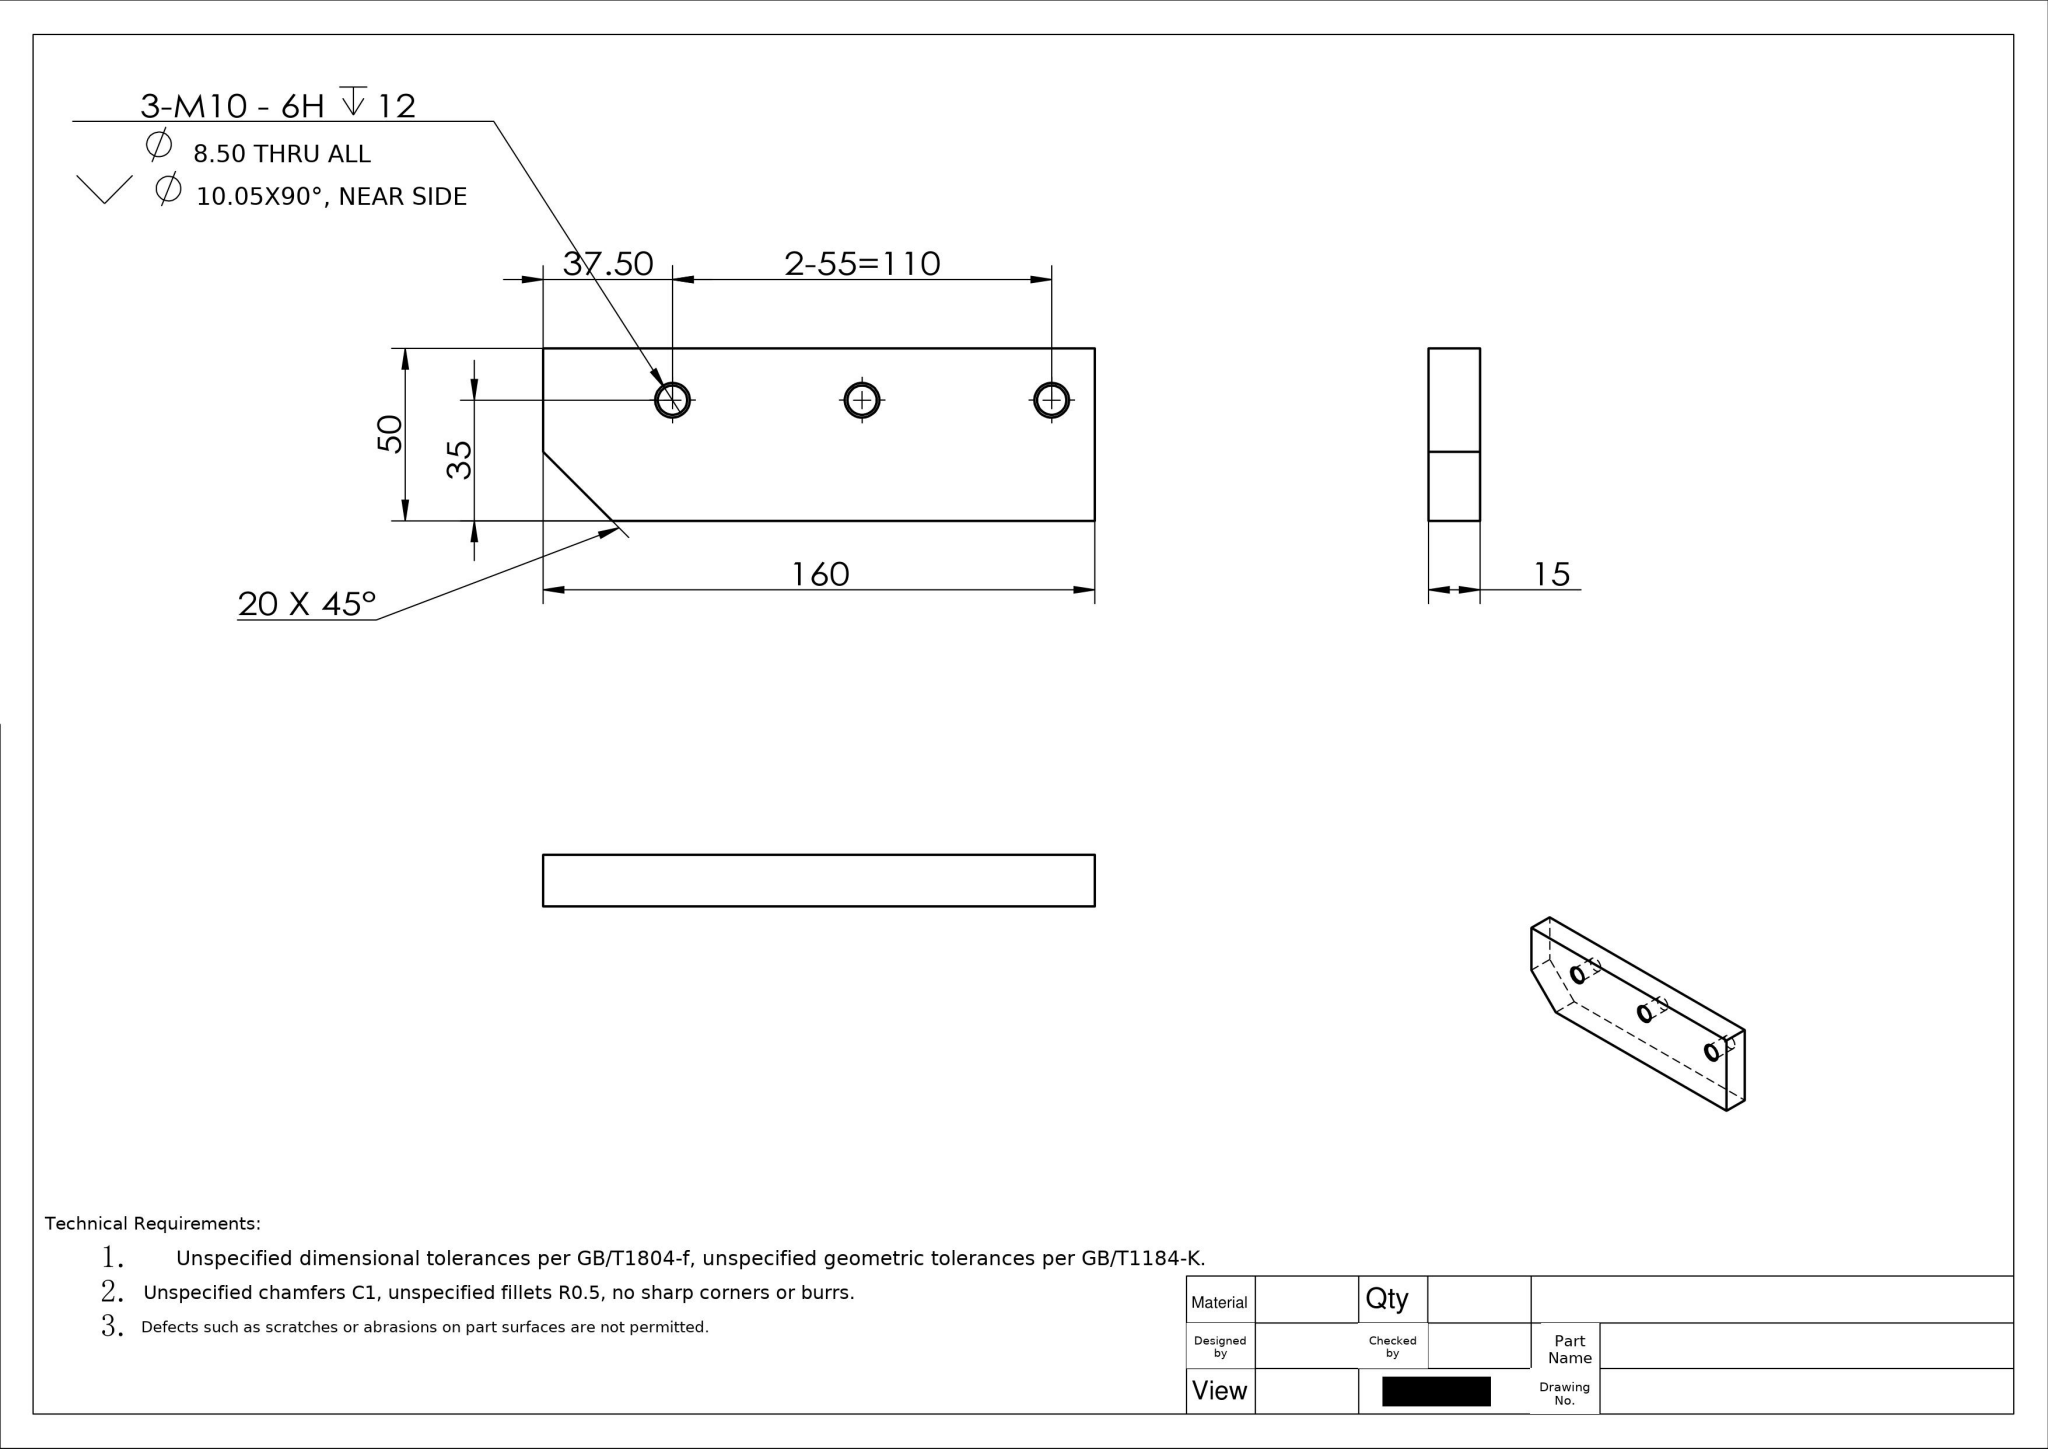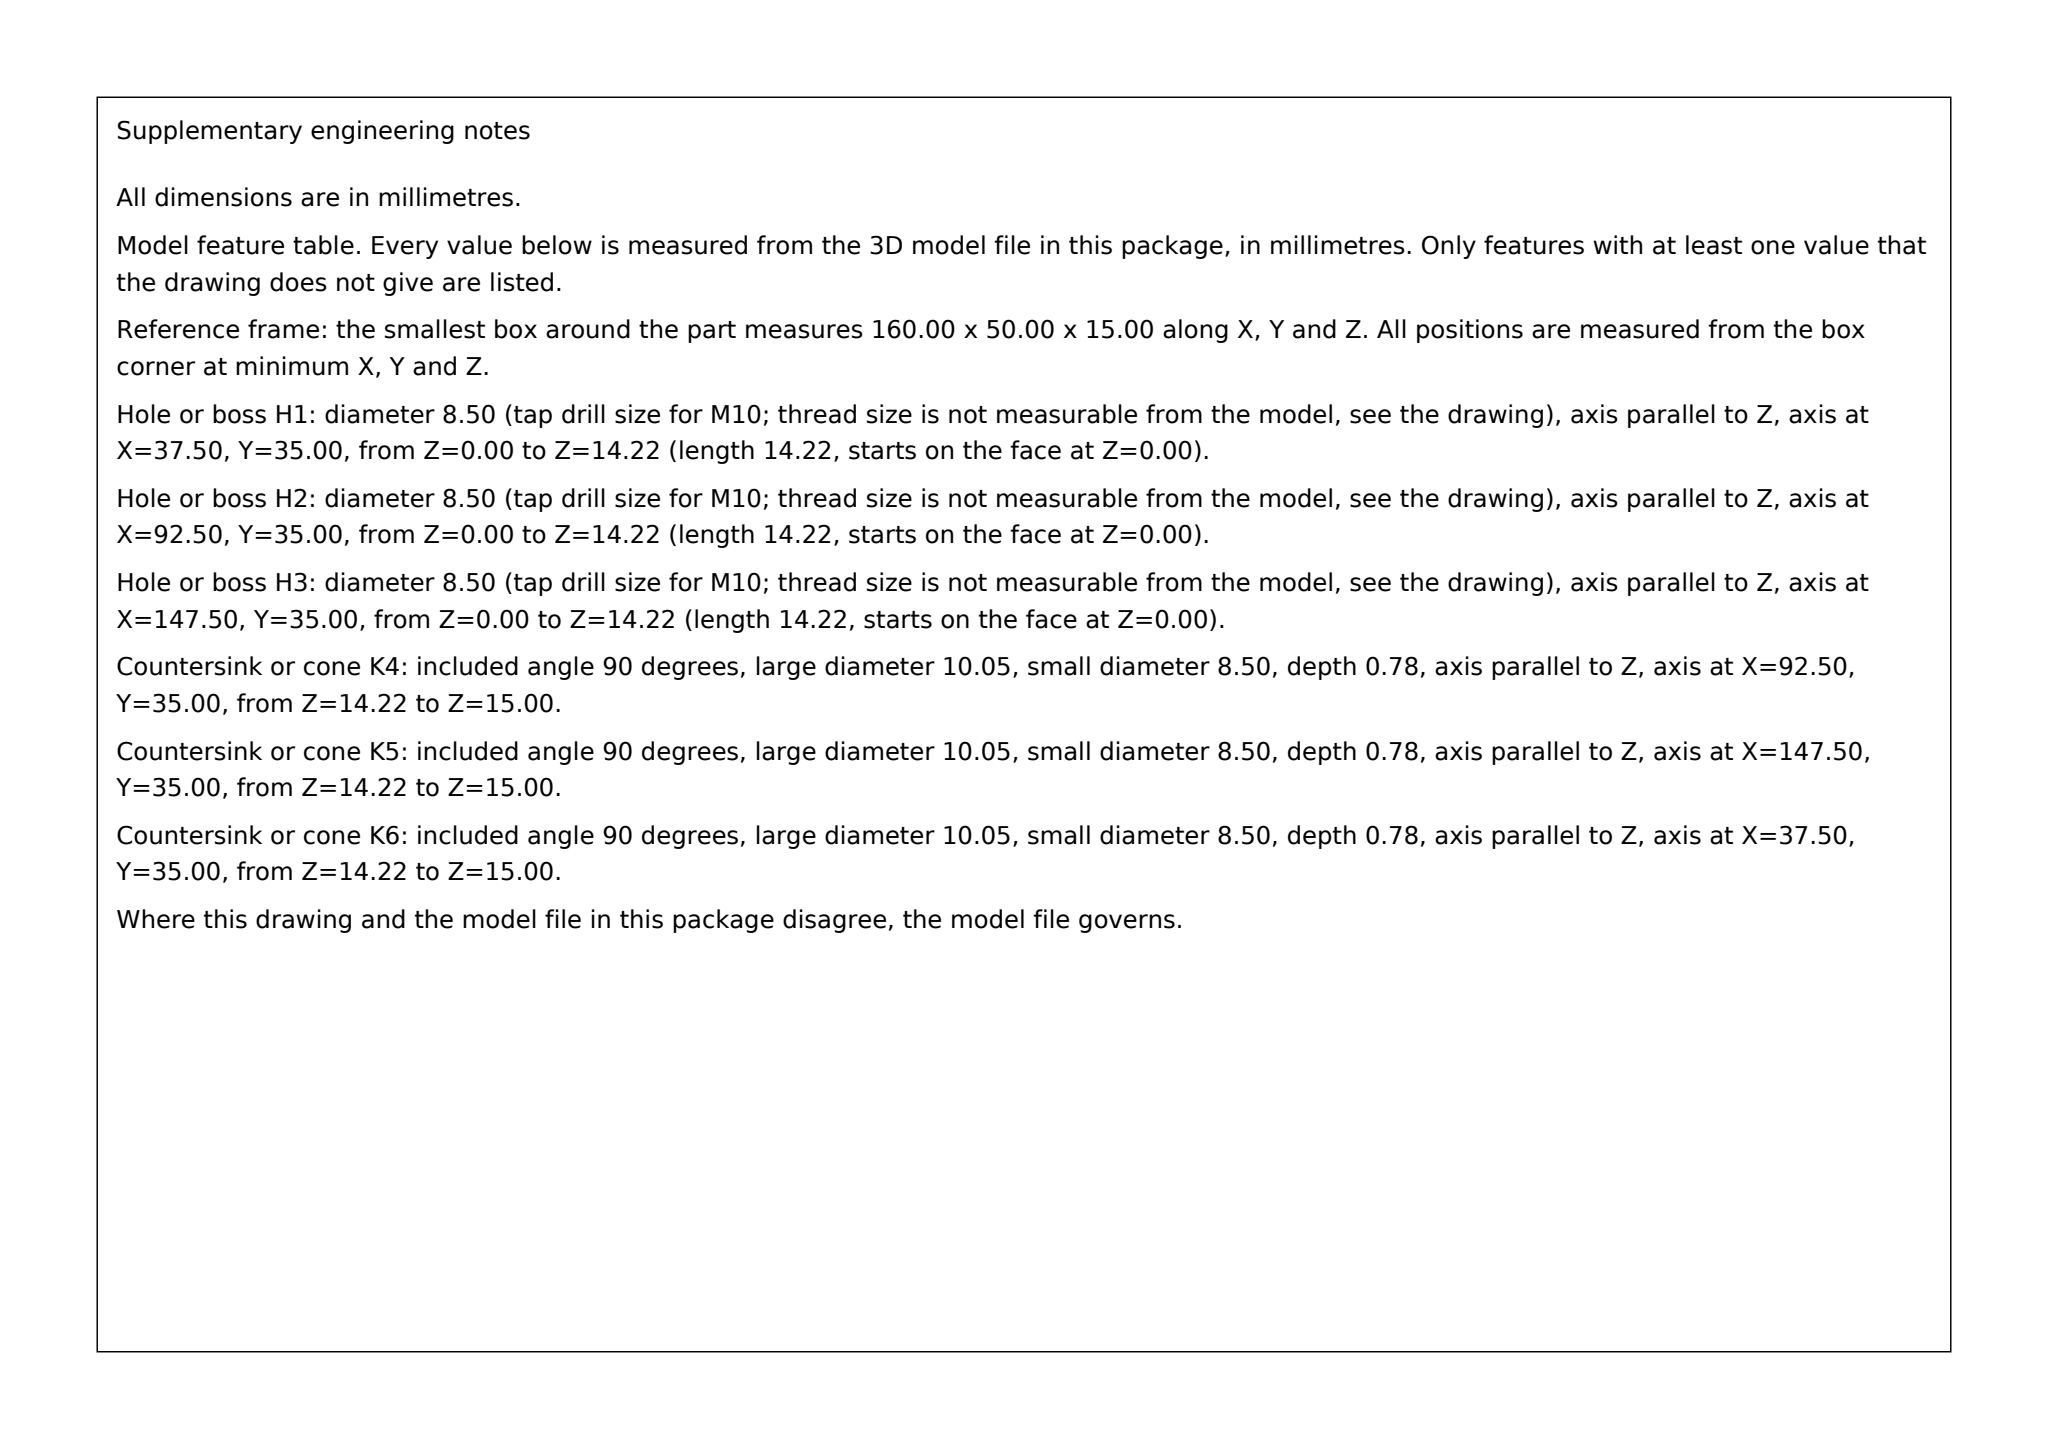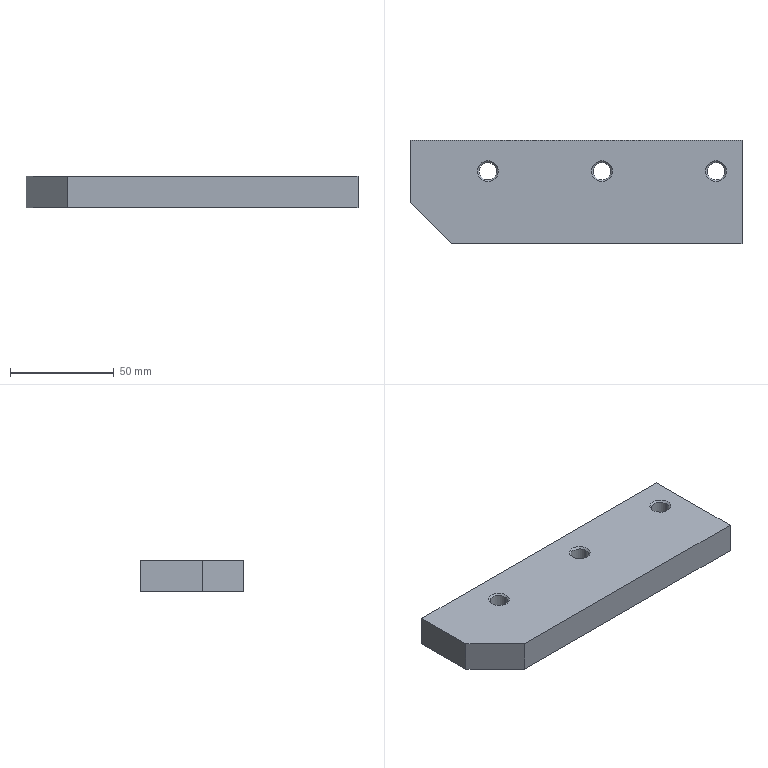Part | SolidWorks | mm | 1 solid | 19 faces | box 160 x 50 x 15 mm | volume 114421 mm3 | plane 7 | cone 6 | cylinder 6 | commonest cylinder face diameters 8.5 x6
build123d program:
from build123d import *

# Parameters (mm, degrees)
SKETCH1_W                    = 160
SKETCH1_H                    = 50
BOSS_EXTRUDE1_DEPTH          = 15
M10_TAPPED_HOLE1_D           = 8.5
M10_TAPPED_HOLE1_CSINK_D     = 10.05
M10_TAPPED_HOLE1_CSINK_ANGLE = 90
CHAMFER1_SIZE                = 20


with BuildPart() as part:
    # Sketch1 → Boss-Extrude1 (new body)
    with BuildSketch(Plane.XY):
        with Locations((80, 25)):
            Rectangle(SKETCH1_W, SKETCH1_H)
    extrude(amount=BOSS_EXTRUDE1_DEPTH)

    # M10 Tapped Hole1 (through all)
    with Locations(Plane.XY.offset(15)):
        with Locations((37.5, 35), (92.5, 35), (147.5, 35)):
            CounterSinkHole(M10_TAPPED_HOLE1_D / 2, M10_TAPPED_HOLE1_CSINK_D / 2, counter_sink_angle=M10_TAPPED_HOLE1_CSINK_ANGLE)

    # Chamfer1
    chamfer1_edges = [part.edges().sort_by_distance(p)[0] for p in [
        (0, 0, 7.5),
    ]]
    chamfer(chamfer1_edges, length=CHAMFER1_SIZE)


solid = part.part
STEP:
#1=CARTESIAN_POINT('',(33.25,35.,14.225));
#2=VERTEX_POINT('',#1);
#3=CARTESIAN_POINT('',(41.75,35.,14.225));
#4=VERTEX_POINT('',#3);
#5=CARTESIAN_POINT('',(37.5,35.,14.225));
#6=DIRECTION('',(0.,0.,1.));
#7=DIRECTION('',(1.,0.,0.));
#8=AXIS2_PLACEMENT_3D('',#5,#6,#7);
#9=CIRCLE('',#8,4.25);
#10=EDGE_CURVE('',#2,#4,#9,.T.);
#11=ORIENTED_EDGE('',*,*,#10,.F.);
#12=CARTESIAN_POINT('',(32.475,35.,15.));
#13=VERTEX_POINT('',#12);
#14=CARTESIAN_POINT('',(32.475,35.,15.));
#15=DIRECTION('',(-0.7071,0.,0.7071));
#16=VECTOR('',#15,1000.);
#17=LINE('',#14,#16);
#18=EDGE_CURVE('',#2,#13,#17,.T.);
#19=ORIENTED_EDGE('',*,*,#18,.T.);
#20=CARTESIAN_POINT('',(42.525,35.,15.));
#21=VERTEX_POINT('',#20);
#22=CARTESIAN_POINT('',(37.5,35.,15.));
#23=DIRECTION('',(0.,0.,1.));
#24=DIRECTION('',(1.,0.,0.));
#25=AXIS2_PLACEMENT_3D('',#22,#23,#24);
#26=CIRCLE('',#25,5.025);
#27=EDGE_CURVE('',#13,#21,#26,.T.);
#28=ORIENTED_EDGE('',*,*,#27,.T.);
#29=CARTESIAN_POINT('',(42.525,35.,15.));
#30=DIRECTION('',(0.7071,0.,0.7071));
#31=VECTOR('',#30,1000.);
#32=LINE('',#29,#31);
#33=EDGE_CURVE('',#4,#21,#32,.T.);
#34=ORIENTED_EDGE('',*,*,#33,.F.);
#35=EDGE_LOOP('',(#11,#19,#28,#34));
#36=FACE_OUTER_BOUND('',#35,.T.);
#37=CARTESIAN_POINT('',(37.5,35.,15.));
#38=DIRECTION('',(0.,0.,1.));
#39=DIRECTION('',(1.,0.,0.));
#40=AXIS2_PLACEMENT_3D('',#37,#38,#39);
#41=CONICAL_SURFACE('',#40,5.025,0.7854);
#42=ADVANCED_FACE('',(#36),#41,.F.);
#43=CARTESIAN_POINT('',(33.25,35.,0.));
#44=VERTEX_POINT('',#43);
#45=CARTESIAN_POINT('',(41.75,35.,0.));
#46=VERTEX_POINT('',#45);
#47=CARTESIAN_POINT('',(37.5,35.,0.));
#48=DIRECTION('',(0.,0.,1.));
#49=DIRECTION('',(1.,0.,0.));
#50=AXIS2_PLACEMENT_3D('',#47,#48,#49);
#51=CIRCLE('',#50,4.25);
#52=EDGE_CURVE('',#44,#46,#51,.T.);
#53=ORIENTED_EDGE('',*,*,#52,.F.);
#54=CARTESIAN_POINT('',(33.25,35.,15.));
#55=DIRECTION('',(0.,0.,1.));
#56=VECTOR('',#55,1000.);
#57=LINE('',#54,#56);
#58=EDGE_CURVE('',#44,#2,#57,.T.);
#59=ORIENTED_EDGE('',*,*,#58,.T.);
#60=ORIENTED_EDGE('',*,*,#10,.T.);
#61=CARTESIAN_POINT('',(41.75,35.,15.));
#62=DIRECTION('',(0.,0.,1.));
#63=VECTOR('',#62,1000.);
#64=LINE('',#61,#63);
#65=EDGE_CURVE('',#46,#4,#64,.T.);
#66=ORIENTED_EDGE('',*,*,#65,.F.);
#67=EDGE_LOOP('',(#53,#59,#60,#66));
#68=FACE_OUTER_BOUND('',#67,.T.);
#69=CARTESIAN_POINT('',(37.5,35.,15.));
#70=DIRECTION('',(0.,0.,1.));
#71=DIRECTION('',(1.,0.,0.));
#72=AXIS2_PLACEMENT_3D('',#69,#70,#71);
#73=CYLINDRICAL_SURFACE('',#72,4.25);
#74=ADVANCED_FACE('',(#68),#73,.F.);
#75=CARTESIAN_POINT('',(88.25,35.,14.225));
#76=VERTEX_POINT('',#75);
#77=CARTESIAN_POINT('',(96.75,35.,14.225));
#78=VERTEX_POINT('',#77);
#79=CARTESIAN_POINT('',(92.5,35.,14.225));
#80=DIRECTION('',(0.,0.,1.));
#81=DIRECTION('',(1.,0.,0.));
#82=AXIS2_PLACEMENT_3D('',#79,#80,#81);
#83=CIRCLE('',#82,4.25);
#84=EDGE_CURVE('',#76,#78,#83,.T.);
#85=ORIENTED_EDGE('',*,*,#84,.F.);
#86=CARTESIAN_POINT('',(87.475,35.,15.));
#87=VERTEX_POINT('',#86);
#88=CARTESIAN_POINT('',(87.475,35.,15.));
#89=DIRECTION('',(-0.7071,0.,0.7071));
#90=VECTOR('',#89,1000.);
#91=LINE('',#88,#90);
#92=EDGE_CURVE('',#76,#87,#91,.T.);
#93=ORIENTED_EDGE('',*,*,#92,.T.);
#94=CARTESIAN_POINT('',(97.525,35.,15.));
#95=VERTEX_POINT('',#94);
#96=CARTESIAN_POINT('',(92.5,35.,15.));
#97=DIRECTION('',(0.,0.,1.));
#98=DIRECTION('',(1.,0.,0.));
#99=AXIS2_PLACEMENT_3D('',#96,#97,#98);
#100=CIRCLE('',#99,5.025);
#101=EDGE_CURVE('',#87,#95,#100,.T.);
#102=ORIENTED_EDGE('',*,*,#101,.T.);
#103=CARTESIAN_POINT('',(97.525,35.,15.));
#104=DIRECTION('',(0.7071,0.,0.7071));
#105=VECTOR('',#104,1000.);
#106=LINE('',#103,#105);
#107=EDGE_CURVE('',#78,#95,#106,.T.);
#108=ORIENTED_EDGE('',*,*,#107,.F.);
#109=EDGE_LOOP('',(#85,#93,#102,#108));
#110=FACE_OUTER_BOUND('',#109,.T.);
#111=CARTESIAN_POINT('',(92.5,35.,15.));
#112=DIRECTION('',(0.,0.,1.));
#113=DIRECTION('',(1.,0.,0.));
#114=AXIS2_PLACEMENT_3D('',#111,#112,#113);
#115=CONICAL_SURFACE('',#114,5.025,0.7854);
#116=ADVANCED_FACE('',(#110),#115,.F.);
#117=CARTESIAN_POINT('',(88.25,35.,0.));
#118=VERTEX_POINT('',#117);
#119=CARTESIAN_POINT('',(96.75,35.,0.));
#120=VERTEX_POINT('',#119);
#121=CARTESIAN_POINT('',(92.5,35.,0.));
#122=DIRECTION('',(0.,0.,1.));
#123=DIRECTION('',(1.,0.,0.));
#124=AXIS2_PLACEMENT_3D('',#121,#122,#123);
#125=CIRCLE('',#124,4.25);
#126=EDGE_CURVE('',#118,#120,#125,.T.);
#127=ORIENTED_EDGE('',*,*,#126,.F.);
#128=CARTESIAN_POINT('',(88.25,35.,15.));
#129=DIRECTION('',(0.,0.,1.));
#130=VECTOR('',#129,1000.);
#131=LINE('',#128,#130);
#132=EDGE_CURVE('',#118,#76,#131,.T.);
#133=ORIENTED_EDGE('',*,*,#132,.T.);
#134=ORIENTED_EDGE('',*,*,#84,.T.);
#135=CARTESIAN_POINT('',(96.75,35.,15.));
#136=DIRECTION('',(0.,0.,1.));
#137=VECTOR('',#136,1000.);
#138=LINE('',#135,#137);
#139=EDGE_CURVE('',#120,#78,#138,.T.);
#140=ORIENTED_EDGE('',*,*,#139,.F.);
#141=EDGE_LOOP('',(#127,#133,#134,#140));
#142=FACE_OUTER_BOUND('',#141,.T.);
#143=CARTESIAN_POINT('',(92.5,35.,15.));
#144=DIRECTION('',(0.,0.,1.));
#145=DIRECTION('',(1.,0.,0.));
#146=AXIS2_PLACEMENT_3D('',#143,#144,#145);
#147=CYLINDRICAL_SURFACE('',#146,4.25);
#148=ADVANCED_FACE('',(#142),#147,.F.);
#149=CARTESIAN_POINT('',(143.25,35.,14.225));
#150=VERTEX_POINT('',#149);
#151=CARTESIAN_POINT('',(151.75,35.,14.225));
#152=VERTEX_POINT('',#151);
#153=CARTESIAN_POINT('',(147.5,35.,14.225));
#154=DIRECTION('',(0.,0.,1.));
#155=DIRECTION('',(1.,0.,0.));
#156=AXIS2_PLACEMENT_3D('',#153,#154,#155);
#157=CIRCLE('',#156,4.25);
#158=EDGE_CURVE('',#150,#152,#157,.T.);
#159=ORIENTED_EDGE('',*,*,#158,.F.);
#160=CARTESIAN_POINT('',(142.475,35.,15.));
#161=VERTEX_POINT('',#160);
#162=CARTESIAN_POINT('',(142.475,35.,15.));
#163=DIRECTION('',(-0.7071,0.,0.7071));
#164=VECTOR('',#163,1000.);
#165=LINE('',#162,#164);
#166=EDGE_CURVE('',#150,#161,#165,.T.);
#167=ORIENTED_EDGE('',*,*,#166,.T.);
#168=CARTESIAN_POINT('',(152.525,35.,15.));
#169=VERTEX_POINT('',#168);
#170=CARTESIAN_POINT('',(147.5,35.,15.));
#171=DIRECTION('',(0.,0.,1.));
#172=DIRECTION('',(1.,0.,0.));
#173=AXIS2_PLACEMENT_3D('',#170,#171,#172);
#174=CIRCLE('',#173,5.025);
#175=EDGE_CURVE('',#161,#169,#174,.T.);
#176=ORIENTED_EDGE('',*,*,#175,.T.);
#177=CARTESIAN_POINT('',(152.525,35.,15.));
#178=DIRECTION('',(0.7071,0.,0.7071));
#179=VECTOR('',#178,1000.);
#180=LINE('',#177,#179);
#181=EDGE_CURVE('',#152,#169,#180,.T.);
#182=ORIENTED_EDGE('',*,*,#181,.F.);
#183=EDGE_LOOP('',(#159,#167,#176,#182));
#184=FACE_OUTER_BOUND('',#183,.T.);
#185=CARTESIAN_POINT('',(147.5,35.,15.));
#186=DIRECTION('',(0.,0.,1.));
#187=DIRECTION('',(1.,0.,0.));
#188=AXIS2_PLACEMENT_3D('',#185,#186,#187);
#189=CONICAL_SURFACE('',#188,5.025,0.7854);
#190=ADVANCED_FACE('',(#184),#189,.F.);
#191=CARTESIAN_POINT('',(143.25,35.,0.));
#192=VERTEX_POINT('',#191);
#193=CARTESIAN_POINT('',(151.75,35.,0.));
#194=VERTEX_POINT('',#193);
#195=CARTESIAN_POINT('',(147.5,35.,0.));
#196=DIRECTION('',(0.,0.,1.));
#197=DIRECTION('',(1.,0.,0.));
#198=AXIS2_PLACEMENT_3D('',#195,#196,#197);
#199=CIRCLE('',#198,4.25);
#200=EDGE_CURVE('',#192,#194,#199,.T.);
#201=ORIENTED_EDGE('',*,*,#200,.F.);
#202=CARTESIAN_POINT('',(143.25,35.,15.));
#203=DIRECTION('',(0.,0.,1.));
#204=VECTOR('',#203,1000.);
#205=LINE('',#202,#204);
#206=EDGE_CURVE('',#192,#150,#205,.T.);
#207=ORIENTED_EDGE('',*,*,#206,.T.);
#208=ORIENTED_EDGE('',*,*,#158,.T.);
#209=CARTESIAN_POINT('',(151.75,35.,15.));
#210=DIRECTION('',(0.,0.,1.));
#211=VECTOR('',#210,1000.);
#212=LINE('',#209,#211);
#213=EDGE_CURVE('',#194,#152,#212,.T.);
#214=ORIENTED_EDGE('',*,*,#213,.F.);
#215=EDGE_LOOP('',(#201,#207,#208,#214));
#216=FACE_OUTER_BOUND('',#215,.T.);
#217=CARTESIAN_POINT('',(147.5,35.,15.));
#218=DIRECTION('',(0.,0.,1.));
#219=DIRECTION('',(1.,0.,0.));
#220=AXIS2_PLACEMENT_3D('',#217,#218,#219);
#221=CYLINDRICAL_SURFACE('',#220,4.25);
#222=ADVANCED_FACE('',(#216),#221,.F.);
#223=CARTESIAN_POINT('',(0.,50.,0.));
#224=VERTEX_POINT('',#223);
#225=CARTESIAN_POINT('',(0.,20.,0.));
#226=VERTEX_POINT('',#225);
#227=CARTESIAN_POINT('',(0.,0.,0.));
#228=DIRECTION('',(0.,-1.,0.));
#229=VECTOR('',#228,1000.);
#230=LINE('',#227,#229);
#231=EDGE_CURVE('',#224,#226,#230,.T.);
#232=ORIENTED_EDGE('',*,*,#231,.T.);
#233=CARTESIAN_POINT('',(0.,20.,15.));
#234=VERTEX_POINT('',#233);
#235=CARTESIAN_POINT('',(0.,20.,15.));
#236=DIRECTION('',(0.,0.,1.));
#237=VECTOR('',#236,1000.);
#238=LINE('',#235,#237);
#239=EDGE_CURVE('',#226,#234,#238,.T.);
#240=ORIENTED_EDGE('',*,*,#239,.T.);
#241=CARTESIAN_POINT('',(0.,50.,15.));
#242=VERTEX_POINT('',#241);
#243=CARTESIAN_POINT('',(0.,0.,15.));
#244=DIRECTION('',(0.,-1.,0.));
#245=VECTOR('',#244,1000.);
#246=LINE('',#243,#245);
#247=EDGE_CURVE('',#242,#234,#246,.T.);
#248=ORIENTED_EDGE('',*,*,#247,.F.);
#249=CARTESIAN_POINT('',(0.,50.,15.));
#250=DIRECTION('',(0.,0.,-1.));
#251=VECTOR('',#250,1000.);
#252=LINE('',#249,#251);
#253=EDGE_CURVE('',#242,#224,#252,.T.);
#254=ORIENTED_EDGE('',*,*,#253,.T.);
#255=EDGE_LOOP('',(#232,#240,#248,#254));
#256=FACE_OUTER_BOUND('',#255,.T.);
#257=CARTESIAN_POINT('',(0.,0.,15.));
#258=DIRECTION('',(1.,0.,0.));
#259=DIRECTION('',(0.,0.,-1.));
#260=AXIS2_PLACEMENT_3D('',#257,#258,#259);
#261=PLANE('',#260);
#262=ADVANCED_FACE('',(#256),#261,.F.);
#263=CARTESIAN_POINT('',(20.,0.,15.));
#264=VERTEX_POINT('',#263);
#265=CARTESIAN_POINT('',(160.,0.,15.));
#266=VERTEX_POINT('',#265);
#267=CARTESIAN_POINT('',(0.,0.,15.));
#268=DIRECTION('',(1.,0.,0.));
#269=VECTOR('',#268,1000.);
#270=LINE('',#267,#269);
#271=EDGE_CURVE('',#264,#266,#270,.T.);
#272=ORIENTED_EDGE('',*,*,#271,.F.);
#273=CARTESIAN_POINT('',(20.,0.,0.));
#274=VERTEX_POINT('',#273);
#275=CARTESIAN_POINT('',(20.,0.,15.));
#276=DIRECTION('',(0.,0.,-1.));
#277=VECTOR('',#276,1000.);
#278=LINE('',#275,#277);
#279=EDGE_CURVE('',#264,#274,#278,.T.);
#280=ORIENTED_EDGE('',*,*,#279,.T.);
#281=CARTESIAN_POINT('',(160.,0.,0.));
#282=VERTEX_POINT('',#281);
#283=CARTESIAN_POINT('',(0.,0.,0.));
#284=DIRECTION('',(1.,0.,0.));
#285=VECTOR('',#284,1000.);
#286=LINE('',#283,#285);
#287=EDGE_CURVE('',#274,#282,#286,.T.);
#288=ORIENTED_EDGE('',*,*,#287,.T.);
#289=CARTESIAN_POINT('',(160.,0.,15.));
#290=DIRECTION('',(0.,0.,-1.));
#291=VECTOR('',#290,1000.);
#292=LINE('',#289,#291);
#293=EDGE_CURVE('',#266,#282,#292,.T.);
#294=ORIENTED_EDGE('',*,*,#293,.F.);
#295=EDGE_LOOP('',(#272,#280,#288,#294));
#296=FACE_OUTER_BOUND('',#295,.T.);
#297=CARTESIAN_POINT('',(0.,0.,15.));
#298=DIRECTION('',(0.,1.,0.));
#299=DIRECTION('',(0.,0.,1.));
#300=AXIS2_PLACEMENT_3D('',#297,#298,#299);
#301=PLANE('',#300);
#302=ADVANCED_FACE('',(#296),#301,.F.);
#303=CARTESIAN_POINT('',(160.,50.,0.));
#304=VERTEX_POINT('',#303);
#305=CARTESIAN_POINT('',(160.,0.,0.));
#306=DIRECTION('',(0.,1.,0.));
#307=VECTOR('',#306,1000.);
#308=LINE('',#305,#307);
#309=EDGE_CURVE('',#282,#304,#308,.T.);
#310=ORIENTED_EDGE('',*,*,#309,.T.);
#311=CARTESIAN_POINT('',(160.,50.,15.));
#312=VERTEX_POINT('',#311);
#313=CARTESIAN_POINT('',(160.,50.,15.));
#314=DIRECTION('',(0.,0.,-1.));
#315=VECTOR('',#314,1000.);
#316=LINE('',#313,#315);
#317=EDGE_CURVE('',#312,#304,#316,.T.);
#318=ORIENTED_EDGE('',*,*,#317,.F.);
#319=CARTESIAN_POINT('',(160.,0.,15.));
#320=DIRECTION('',(0.,1.,0.));
#321=VECTOR('',#320,1000.);
#322=LINE('',#319,#321);
#323=EDGE_CURVE('',#266,#312,#322,.T.);
#324=ORIENTED_EDGE('',*,*,#323,.F.);
#325=ORIENTED_EDGE('',*,*,#293,.T.);
#326=EDGE_LOOP('',(#310,#318,#324,#325));
#327=FACE_OUTER_BOUND('',#326,.T.);
#328=CARTESIAN_POINT('',(160.,0.,15.));
#329=DIRECTION('',(-1.,0.,0.));
#330=DIRECTION('',(0.,0.,1.));
#331=AXIS2_PLACEMENT_3D('',#328,#329,#330);
#332=PLANE('',#331);
#333=ADVANCED_FACE('',(#327),#332,.F.);
#334=CARTESIAN_POINT('',(0.,50.,0.));
#335=DIRECTION('',(-1.,0.,0.));
#336=VECTOR('',#335,1000.);
#337=LINE('',#334,#336);
#338=EDGE_CURVE('',#304,#224,#337,.T.);
#339=ORIENTED_EDGE('',*,*,#338,.T.);
#340=ORIENTED_EDGE('',*,*,#253,.F.);
#341=CARTESIAN_POINT('',(0.,50.,15.));
#342=DIRECTION('',(-1.,0.,0.));
#343=VECTOR('',#342,1000.);
#344=LINE('',#341,#343);
#345=EDGE_CURVE('',#312,#242,#344,.T.);
#346=ORIENTED_EDGE('',*,*,#345,.F.);
#347=ORIENTED_EDGE('',*,*,#317,.T.);
#348=EDGE_LOOP('',(#339,#340,#346,#347));
#349=FACE_OUTER_BOUND('',#348,.T.);
#350=CARTESIAN_POINT('',(0.,50.,15.));
#351=DIRECTION('',(0.,-1.,0.));
#352=DIRECTION('',(0.,0.,-1.));
#353=AXIS2_PLACEMENT_3D('',#350,#351,#352);
#354=PLANE('',#353);
#355=ADVANCED_FACE('',(#349),#354,.F.);
#356=CARTESIAN_POINT('',(37.5,35.,15.));
#357=DIRECTION('',(0.,0.,1.));
#358=DIRECTION('',(1.,0.,0.));
#359=AXIS2_PLACEMENT_3D('',#356,#357,#358);
#360=CIRCLE('',#359,5.025);
#361=EDGE_CURVE('',#21,#13,#360,.T.);
#362=ORIENTED_EDGE('',*,*,#361,.F.);
#363=ORIENTED_EDGE('',*,*,#27,.F.);
#364=EDGE_LOOP('',(#362,#363));
#365=FACE_BOUND('',#364,.T.);
#366=CARTESIAN_POINT('',(92.5,35.,15.));
#367=DIRECTION('',(0.,0.,1.));
#368=DIRECTION('',(1.,0.,0.));
#369=AXIS2_PLACEMENT_3D('',#366,#367,#368);
#370=CIRCLE('',#369,5.025);
#371=EDGE_CURVE('',#95,#87,#370,.T.);
#372=ORIENTED_EDGE('',*,*,#371,.F.);
#373=ORIENTED_EDGE('',*,*,#101,.F.);
#374=EDGE_LOOP('',(#372,#373));
#375=FACE_BOUND('',#374,.T.);
#376=CARTESIAN_POINT('',(147.5,35.,15.));
#377=DIRECTION('',(0.,0.,1.));
#378=DIRECTION('',(1.,0.,0.));
#379=AXIS2_PLACEMENT_3D('',#376,#377,#378);
#380=CIRCLE('',#379,5.025);
#381=EDGE_CURVE('',#169,#161,#380,.T.);
#382=ORIENTED_EDGE('',*,*,#381,.F.);
#383=ORIENTED_EDGE('',*,*,#175,.F.);
#384=EDGE_LOOP('',(#382,#383));
#385=FACE_BOUND('',#384,.T.);
#386=ORIENTED_EDGE('',*,*,#247,.T.);
#387=CARTESIAN_POINT('',(20.,0.,15.));
#388=DIRECTION('',(0.7071,-0.7071,0.));
#389=VECTOR('',#388,1000.);
#390=LINE('',#387,#389);
#391=EDGE_CURVE('',#234,#264,#390,.T.);
#392=ORIENTED_EDGE('',*,*,#391,.T.);
#393=ORIENTED_EDGE('',*,*,#271,.T.);
#394=ORIENTED_EDGE('',*,*,#323,.T.);
#395=ORIENTED_EDGE('',*,*,#345,.T.);
#396=EDGE_LOOP('',(#386,#392,#393,#394,#395));
#397=FACE_OUTER_BOUND('',#396,.T.);
#398=CARTESIAN_POINT('',(0.,0.,15.));
#399=DIRECTION('',(0.,0.,-1.));
#400=DIRECTION('',(-1.,0.,0.));
#401=AXIS2_PLACEMENT_3D('',#398,#399,#400);
#402=PLANE('',#401);
#403=ADVANCED_FACE('',(#365,#375,#385,#397),#402,.F.);
#404=CARTESIAN_POINT('',(37.5,35.,0.));
#405=DIRECTION('',(0.,0.,1.));
#406=DIRECTION('',(1.,0.,0.));
#407=AXIS2_PLACEMENT_3D('',#404,#405,#406);
#408=CIRCLE('',#407,4.25);
#409=EDGE_CURVE('',#46,#44,#408,.T.);
#410=ORIENTED_EDGE('',*,*,#409,.T.);
#411=ORIENTED_EDGE('',*,*,#52,.T.);
#412=EDGE_LOOP('',(#410,#411));
#413=FACE_BOUND('',#412,.T.);
#414=CARTESIAN_POINT('',(92.5,35.,0.));
#415=DIRECTION('',(0.,0.,1.));
#416=DIRECTION('',(1.,0.,0.));
#417=AXIS2_PLACEMENT_3D('',#414,#415,#416);
#418=CIRCLE('',#417,4.25);
#419=EDGE_CURVE('',#120,#118,#418,.T.);
#420=ORIENTED_EDGE('',*,*,#419,.T.);
#421=ORIENTED_EDGE('',*,*,#126,.T.);
#422=EDGE_LOOP('',(#420,#421));
#423=FACE_BOUND('',#422,.T.);
#424=CARTESIAN_POINT('',(147.5,35.,0.));
#425=DIRECTION('',(0.,0.,1.));
#426=DIRECTION('',(1.,0.,0.));
#427=AXIS2_PLACEMENT_3D('',#424,#425,#426);
#428=CIRCLE('',#427,4.25);
#429=EDGE_CURVE('',#194,#192,#428,.T.);
#430=ORIENTED_EDGE('',*,*,#429,.T.);
#431=ORIENTED_EDGE('',*,*,#200,.T.);
#432=EDGE_LOOP('',(#430,#431));
#433=FACE_BOUND('',#432,.T.);
#434=ORIENTED_EDGE('',*,*,#287,.F.);
#435=CARTESIAN_POINT('',(10.,10.,0.));
#436=DIRECTION('',(-0.7071,0.7071,0.));
#437=VECTOR('',#436,1000.);
#438=LINE('',#435,#437);
#439=EDGE_CURVE('',#274,#226,#438,.T.);
#440=ORIENTED_EDGE('',*,*,#439,.T.);
#441=ORIENTED_EDGE('',*,*,#231,.F.);
#442=ORIENTED_EDGE('',*,*,#338,.F.);
#443=ORIENTED_EDGE('',*,*,#309,.F.);
#444=EDGE_LOOP('',(#434,#440,#441,#442,#443));
#445=FACE_OUTER_BOUND('',#444,.T.);
#446=CARTESIAN_POINT('',(0.,0.,0.));
#447=DIRECTION('',(0.,0.,-1.));
#448=DIRECTION('',(-1.,0.,0.));
#449=AXIS2_PLACEMENT_3D('',#446,#447,#448);
#450=PLANE('',#449);
#451=ADVANCED_FACE('',(#413,#423,#433,#445),#450,.T.);
#452=ORIENTED_EDGE('',*,*,#206,.F.);
#453=ORIENTED_EDGE('',*,*,#429,.F.);
#454=ORIENTED_EDGE('',*,*,#213,.T.);
#455=CARTESIAN_POINT('',(147.5,35.,14.225));
#456=DIRECTION('',(0.,0.,1.));
#457=DIRECTION('',(1.,0.,0.));
#458=AXIS2_PLACEMENT_3D('',#455,#456,#457);
#459=CIRCLE('',#458,4.25);
#460=EDGE_CURVE('',#152,#150,#459,.T.);
#461=ORIENTED_EDGE('',*,*,#460,.T.);
#462=EDGE_LOOP('',(#452,#453,#454,#461));
#463=FACE_OUTER_BOUND('',#462,.T.);
#464=CARTESIAN_POINT('',(147.5,35.,15.));
#465=DIRECTION('',(0.,0.,1.));
#466=DIRECTION('',(1.,0.,0.));
#467=AXIS2_PLACEMENT_3D('',#464,#465,#466);
#468=CYLINDRICAL_SURFACE('',#467,4.25);
#469=ADVANCED_FACE('',(#463),#468,.F.);
#470=ORIENTED_EDGE('',*,*,#166,.F.);
#471=ORIENTED_EDGE('',*,*,#460,.F.);
#472=ORIENTED_EDGE('',*,*,#181,.T.);
#473=ORIENTED_EDGE('',*,*,#381,.T.);
#474=EDGE_LOOP('',(#470,#471,#472,#473));
#475=FACE_OUTER_BOUND('',#474,.T.);
#476=CARTESIAN_POINT('',(147.5,35.,15.));
#477=DIRECTION('',(0.,0.,1.));
#478=DIRECTION('',(1.,0.,0.));
#479=AXIS2_PLACEMENT_3D('',#476,#477,#478);
#480=CONICAL_SURFACE('',#479,5.025,0.7854);
#481=ADVANCED_FACE('',(#475),#480,.F.);
#482=ORIENTED_EDGE('',*,*,#132,.F.);
#483=ORIENTED_EDGE('',*,*,#419,.F.);
#484=ORIENTED_EDGE('',*,*,#139,.T.);
#485=CARTESIAN_POINT('',(92.5,35.,14.225));
#486=DIRECTION('',(0.,0.,1.));
#487=DIRECTION('',(1.,0.,0.));
#488=AXIS2_PLACEMENT_3D('',#485,#486,#487);
#489=CIRCLE('',#488,4.25);
#490=EDGE_CURVE('',#78,#76,#489,.T.);
#491=ORIENTED_EDGE('',*,*,#490,.T.);
#492=EDGE_LOOP('',(#482,#483,#484,#491));
#493=FACE_OUTER_BOUND('',#492,.T.);
#494=CARTESIAN_POINT('',(92.5,35.,15.));
#495=DIRECTION('',(0.,0.,1.));
#496=DIRECTION('',(1.,0.,0.));
#497=AXIS2_PLACEMENT_3D('',#494,#495,#496);
#498=CYLINDRICAL_SURFACE('',#497,4.25);
#499=ADVANCED_FACE('',(#493),#498,.F.);
#500=ORIENTED_EDGE('',*,*,#92,.F.);
#501=ORIENTED_EDGE('',*,*,#490,.F.);
#502=ORIENTED_EDGE('',*,*,#107,.T.);
#503=ORIENTED_EDGE('',*,*,#371,.T.);
#504=EDGE_LOOP('',(#500,#501,#502,#503));
#505=FACE_OUTER_BOUND('',#504,.T.);
#506=CARTESIAN_POINT('',(92.5,35.,15.));
#507=DIRECTION('',(0.,0.,1.));
#508=DIRECTION('',(1.,0.,0.));
#509=AXIS2_PLACEMENT_3D('',#506,#507,#508);
#510=CONICAL_SURFACE('',#509,5.025,0.7854);
#511=ADVANCED_FACE('',(#505),#510,.F.);
#512=ORIENTED_EDGE('',*,*,#58,.F.);
#513=ORIENTED_EDGE('',*,*,#409,.F.);
#514=ORIENTED_EDGE('',*,*,#65,.T.);
#515=CARTESIAN_POINT('',(37.5,35.,14.225));
#516=DIRECTION('',(0.,0.,1.));
#517=DIRECTION('',(1.,0.,0.));
#518=AXIS2_PLACEMENT_3D('',#515,#516,#517);
#519=CIRCLE('',#518,4.25);
#520=EDGE_CURVE('',#4,#2,#519,.T.);
#521=ORIENTED_EDGE('',*,*,#520,.T.);
#522=EDGE_LOOP('',(#512,#513,#514,#521));
#523=FACE_OUTER_BOUND('',#522,.T.);
#524=CARTESIAN_POINT('',(37.5,35.,15.));
#525=DIRECTION('',(0.,0.,1.));
#526=DIRECTION('',(1.,0.,0.));
#527=AXIS2_PLACEMENT_3D('',#524,#525,#526);
#528=CYLINDRICAL_SURFACE('',#527,4.25);
#529=ADVANCED_FACE('',(#523),#528,.F.);
#530=ORIENTED_EDGE('',*,*,#18,.F.);
#531=ORIENTED_EDGE('',*,*,#520,.F.);
#532=ORIENTED_EDGE('',*,*,#33,.T.);
#533=ORIENTED_EDGE('',*,*,#361,.T.);
#534=EDGE_LOOP('',(#530,#531,#532,#533));
#535=FACE_OUTER_BOUND('',#534,.T.);
#536=CARTESIAN_POINT('',(37.5,35.,15.));
#537=DIRECTION('',(0.,0.,1.));
#538=DIRECTION('',(1.,0.,0.));
#539=AXIS2_PLACEMENT_3D('',#536,#537,#538);
#540=CONICAL_SURFACE('',#539,5.025,0.7854);
#541=ADVANCED_FACE('',(#535),#540,.F.);
#542=ORIENTED_EDGE('',*,*,#391,.F.);
#543=ORIENTED_EDGE('',*,*,#239,.F.);
#544=ORIENTED_EDGE('',*,*,#439,.F.);
#545=ORIENTED_EDGE('',*,*,#279,.F.);
#546=EDGE_LOOP('',(#542,#543,#544,#545));
#547=FACE_OUTER_BOUND('',#546,.T.);
#548=CARTESIAN_POINT('',(20.,0.,15.));
#549=DIRECTION('',(0.7071,0.7071,0.));
#550=DIRECTION('',(0.,0.,-1.));
#551=AXIS2_PLACEMENT_3D('',#548,#549,#550);
#552=PLANE('',#551);
#553=ADVANCED_FACE('',(#547),#552,.F.);
#554=CLOSED_SHELL('',(#42,#74,#116,#148,#190,#222,#262,#302,#333,#355,#403,#451,#469,#481,#499,#511,#529,#541,#553));
#555=MANIFOLD_SOLID_BREP('',#554);
#556=CARTESIAN_POINT('',(0.,0.,0.));
#557=DIRECTION('',(0.,0.,1.));
#558=DIRECTION('',(1.,0.,0.));
#559=AXIS2_PLACEMENT_3D('',#556,#557,#558);
#560=(LENGTH_UNIT()NAMED_UNIT(*)SI_UNIT(.MILLI.,.METRE.));
#561=UNCERTAINTY_MEASURE_WITH_UNIT(LENGTH_MEASURE(0.00001),#560,'','');
#562=(NAMED_UNIT(*)PLANE_ANGLE_UNIT()SI_UNIT($,.RADIAN.));
#563=(NAMED_UNIT(*)SI_UNIT($,.STERADIAN.)SOLID_ANGLE_UNIT());
#564=(GEOMETRIC_REPRESENTATION_CONTEXT(3)GLOBAL_UNCERTAINTY_ASSIGNED_CONTEXT((#561))GLOBAL_UNIT_ASSIGNED_CONTEXT((#560,#562,#563))REPRESENTATION_CONTEXT('',''));
#565=ADVANCED_BREP_SHAPE_REPRESENTATION('',(#555,#559),#564);